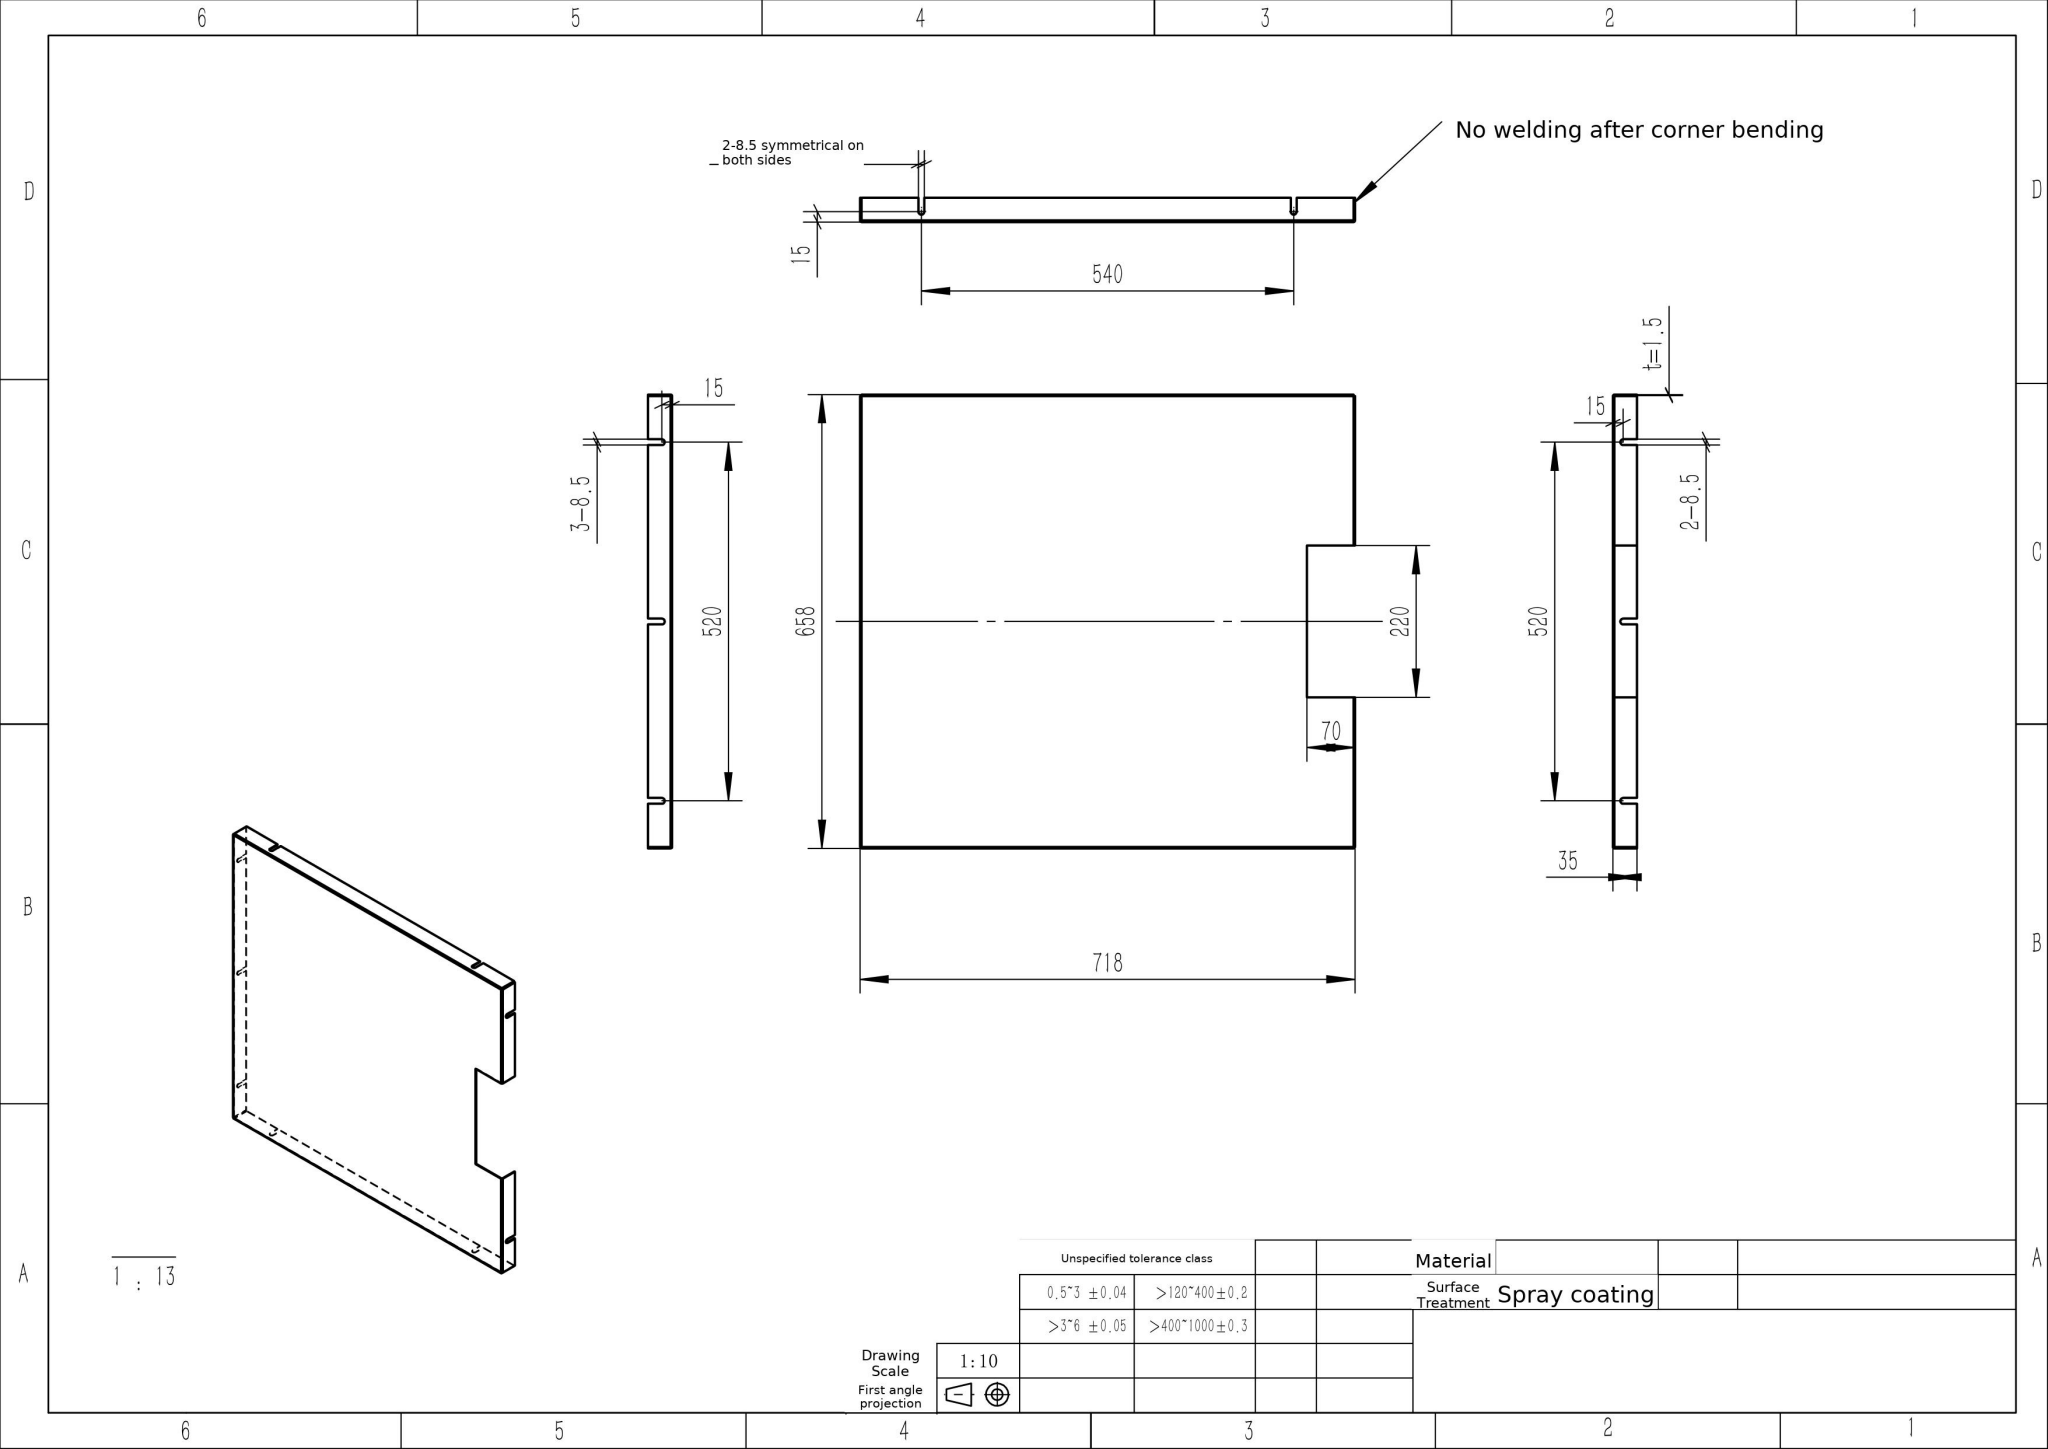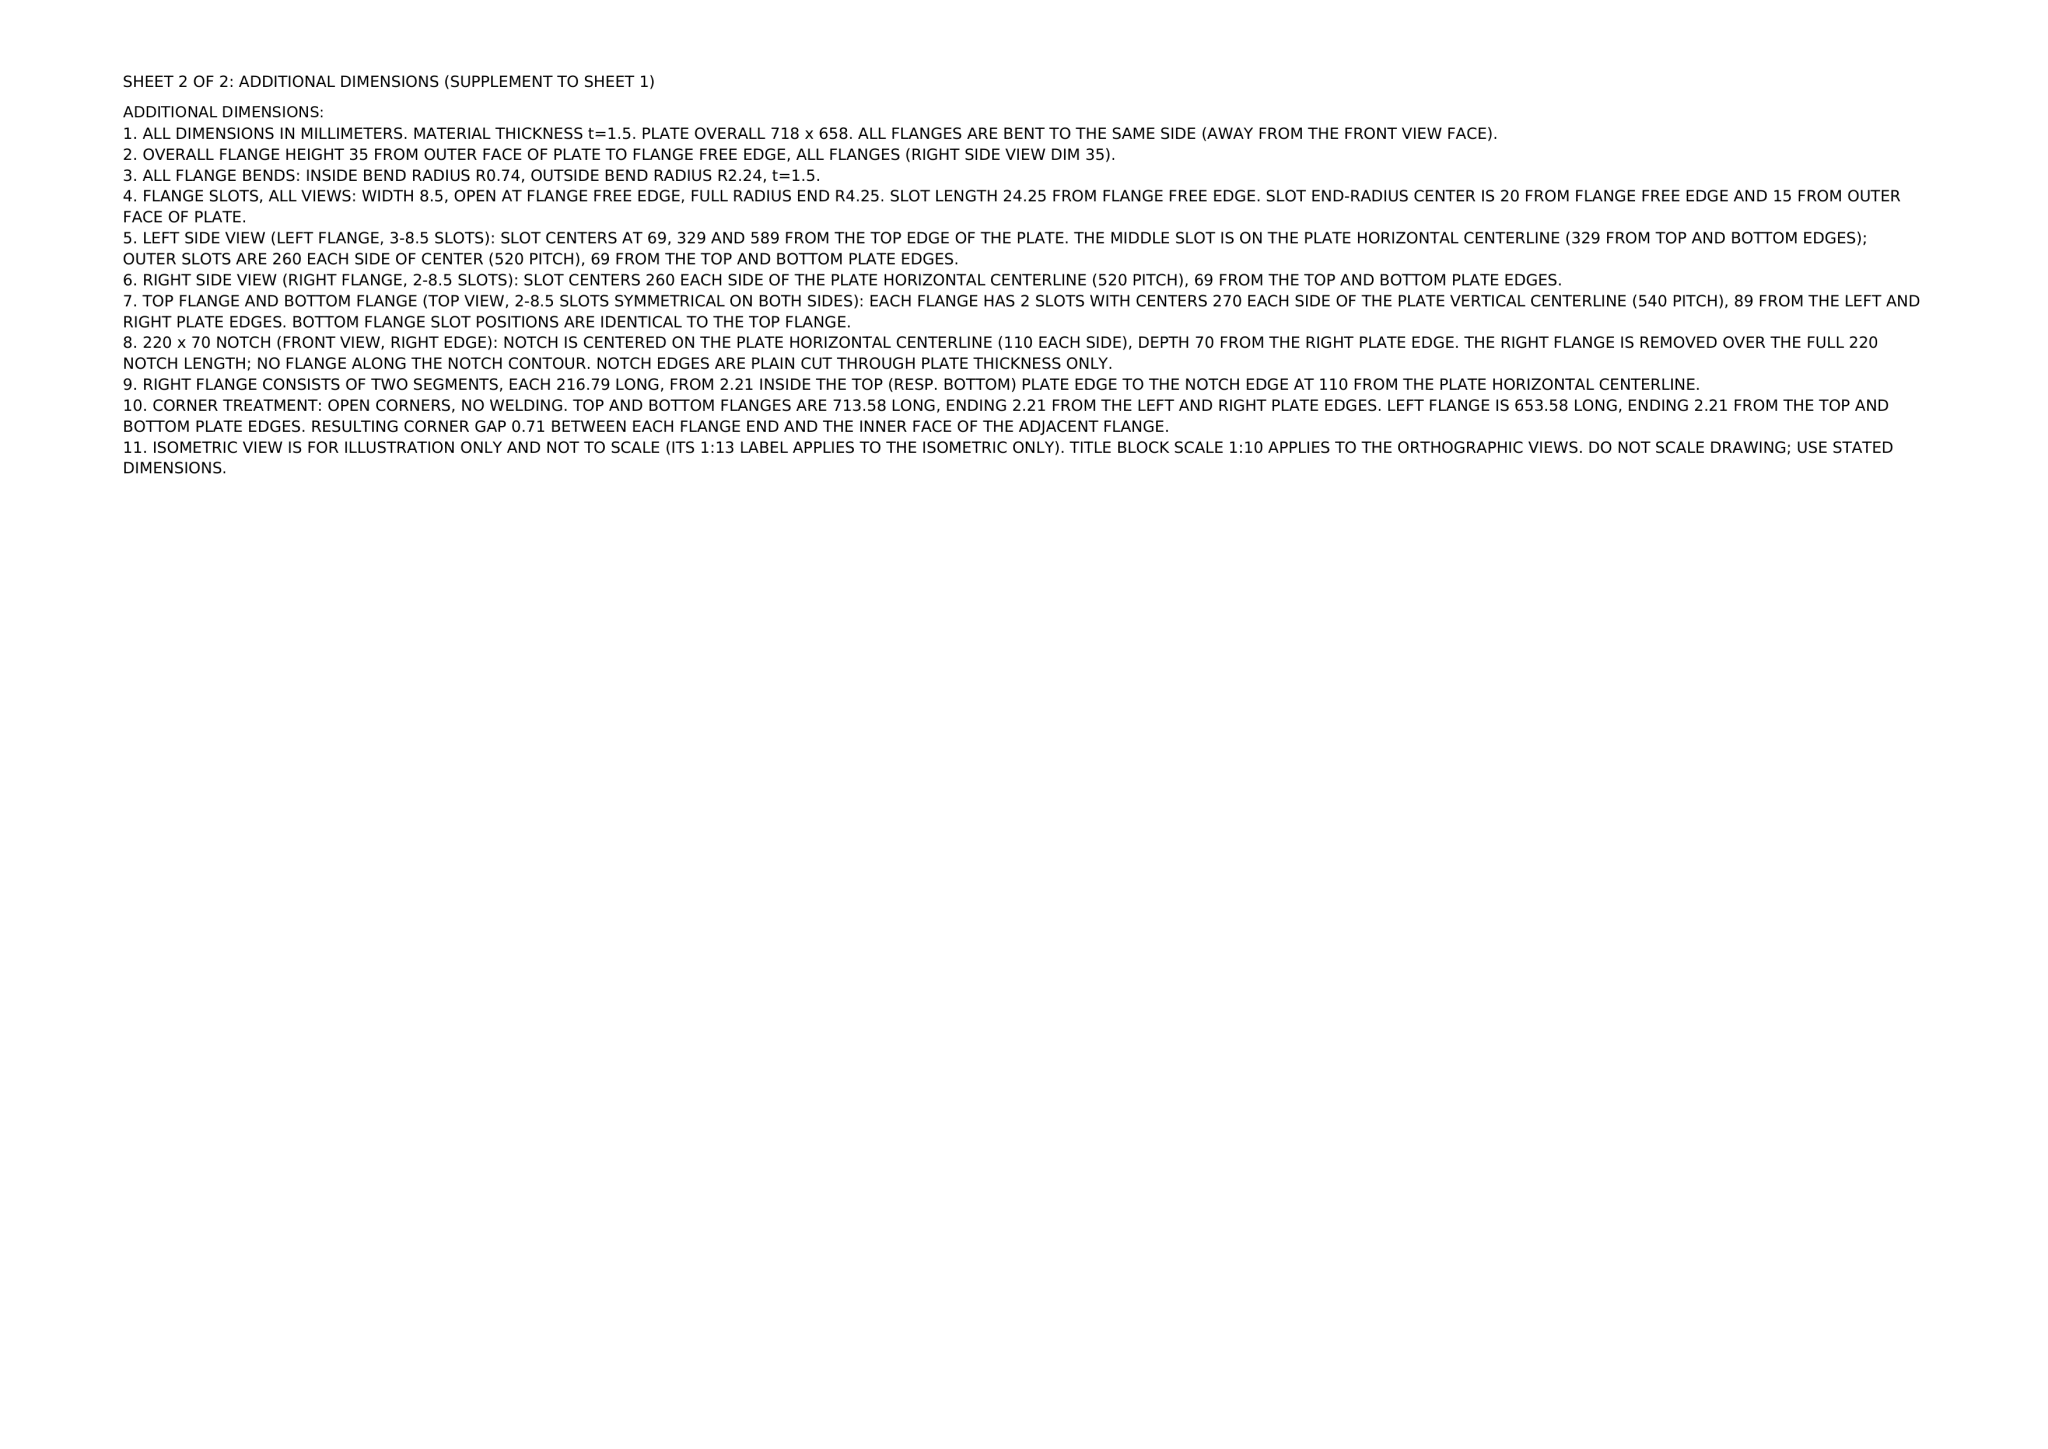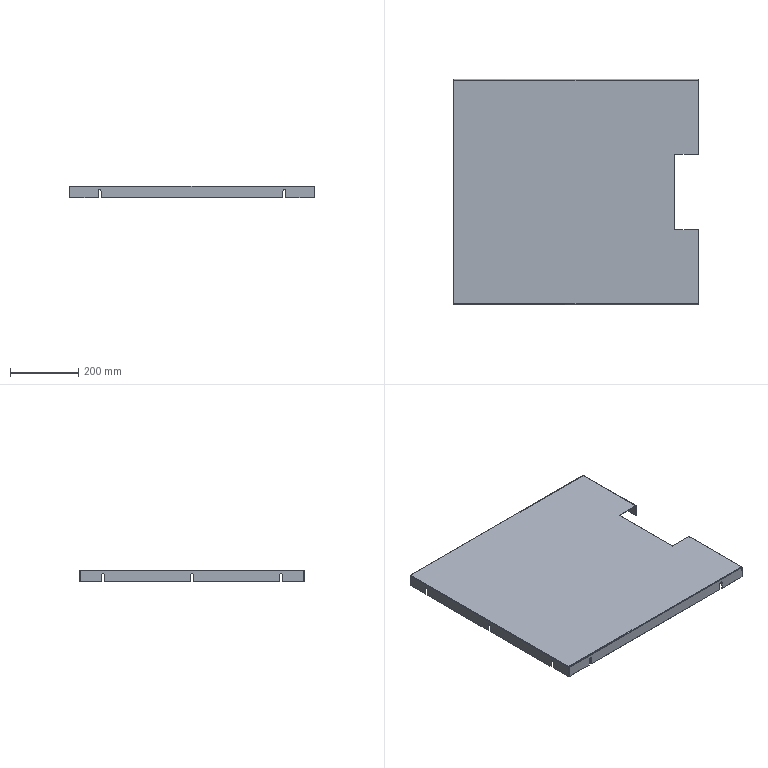Part | NX | mm | 1 solid | 90 faces | box 718 x 658 x 35 mm | volume 806798 mm3 | plane 59 | cylinder 23 | spline 8 | commonest cylinder face diameters 8.5 x13 4.473 x5 1.473 x5